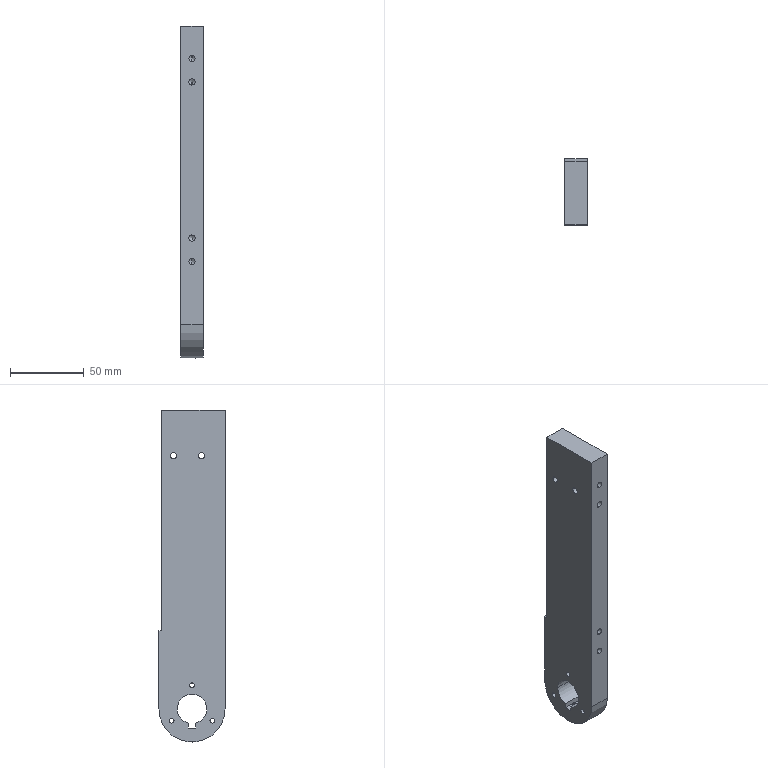Component | SolidWorks | 04-1 | 1 solid | 54 faces | box 15 x 45 x 225.5 mm | volume 137244 mm3 | cylinder 30 | cone 14 | plane 10 | commonest cylinder face diameters 4.2 x20 3.3 x6 20 x3 45 x1
build123d program:
from build123d import *

# Parameters (mm, degrees)
SKETCH1_W             = 203
SKETCH1_H             = 45
EXTRUDE1_DEPTH        = 7.5
SKETCH2_R             = 22.5
EXTRUDE2_DEPTH        = 15
SKETCH4_R             = 10
EXTRUDE3_DEPTH        = 127.914
SKETCH5_W             = 150
SKETCH5_H             = 15
CUT_EXTRUDE1_DEPTH    = 2
SKETCH6_W             = 7
SKETCH6_H             = 5
EXTRUDE4_DEPTH        = 127.914
M5_TAPPED_HOLE1_D     = 4.2
M5_TAPPED_HOLE1_DEPTH = 14
M5_TAPPED_HOLE1_TIP   = 1.262
M5_TAPPED_HOLE2_D     = 4.2
M5_TAPPED_HOLE2_DEPTH = 14
M5_TAPPED_HOLE2_TIP   = 1.262
M4_TAPPED_HOLE1_D     = 3.3
M5_TAPPED_HOLE3_D     = 4.2
M5_TAPPED_HOLE4_D     = 4.2
M5_TAPPED_HOLE4_DEPTH = 12.4
M5_TAPPED_HOLE4_TIP   = 1.262


with BuildPart() as part:
    # Sketch1 → Extrude1 (new, symmetric)
    with BuildSketch(Plane(origin=(0, 0, 0), x_dir=(1, 0, 0), z_dir=(0, 1, 0))):
        Rectangle(SKETCH1_W, SKETCH1_H)
    extrude(amount=EXTRUDE1_DEPTH, both=True)

    # Sketch2 → Extrude2 (add)
    with BuildSketch(Plane(origin=(0, 7.5, 0), x_dir=(1, 0, 0), z_dir=(0, 1, 0))):
        with Locations((101.5, 0)):
            Circle(SKETCH2_R)
    extrude(amount=-EXTRUDE2_DEPTH)

    # Sketch4 → Extrude3 (cut, through all)
    with BuildSketch(Plane(origin=(0, 7.5, 0), x_dir=(1, 0, 0), z_dir=(0, 1, 0))):
        with Locations(Location((101.5, 0, 0), (0, 0, 270))):
            Circle(SKETCH4_R)
    extrude(amount=-EXTRUDE3_DEPTH, mode=Mode.SUBTRACT)

    # Sketch5 → Cut-Extrude1 (cut)
    with BuildSketch(Plane(origin=(0, 0, -22.5), x_dir=(-1, 0, 0), z_dir=(0, 0, -1))):
        with Locations((26.5, 0)):
            Rectangle(SKETCH5_W, SKETCH5_H)
    extrude(amount=-CUT_EXTRUDE1_DEPTH, mode=Mode.SUBTRACT)

    # Sketch6 → Extrude4 (cut, through all)
    with BuildSketch(Plane(origin=(0, 7.5, 0), x_dir=(1, 0, 0), z_dir=(0, 1, 0))):
        with Locations((111, 0)):
            Rectangle(SKETCH6_W, SKETCH6_H)
    extrude(amount=-EXTRUDE4_DEPTH, mode=Mode.SUBTRACT)

    # M5 Tapped Hole1
    with Locations(Plane.XY.offset(22.5)):
        with Locations((-79.5, 0), (-63.5, 0), (42.5, 0), (58.5, 0)):
            Hole(M5_TAPPED_HOLE1_D / 2, depth=M5_TAPPED_HOLE1_DEPTH)
            with Locations((0, 0, -(M5_TAPPED_HOLE1_DEPTH + M5_TAPPED_HOLE1_TIP / 2))):  # 118° drill point
                Cone(0, M5_TAPPED_HOLE1_D / 2, M5_TAPPED_HOLE1_TIP, mode=Mode.SUBTRACT)

    # M5 Tapped Hole2
    with Locations(Plane.ZY.offset(-114.5)):
        with Locations((0, 0)):
            Hole(M5_TAPPED_HOLE2_D / 2, depth=M5_TAPPED_HOLE2_DEPTH)
            with Locations((0, 0, -(M5_TAPPED_HOLE2_DEPTH + M5_TAPPED_HOLE2_TIP / 2))):  # 118° drill point
                Cone(0, M5_TAPPED_HOLE2_D / 2, M5_TAPPED_HOLE2_TIP, mode=Mode.SUBTRACT)

    # M4 Tapped Hole1 (through all)
    with Locations(Plane(origin=(0, 7.5, 0), x_dir=(1, 0, 0), z_dir=(0, 1, 0))):
        with Locations((85.5, 0), (109.5, 13.856), (109.5, -13.856)):
            Hole(M4_TAPPED_HOLE1_D / 2)

    # M5 Tapped Hole3 (through all)
    with Locations(Plane(origin=(0, -7.5, 0), x_dir=(-1, 0, 0), z_dir=(0, -1, 0))):
        with Locations((70.5, 12.5), (70.5, -6.5)):
            Hole(M5_TAPPED_HOLE3_D / 2)

    # M5 Tapped Hole4
    with Locations(Plane(origin=(0, 0, -20.5), x_dir=(-1, 0, 0), z_dir=(0, 0, -1))):
        with Locations((86.5, 0), (26.5, 0), (-33.5, 0), (86.5, -156), (26.5, -156), (-33.5, -156)):
            Hole(M5_TAPPED_HOLE4_D / 2, depth=M5_TAPPED_HOLE4_DEPTH)
            with Locations((0, 0, -(M5_TAPPED_HOLE4_DEPTH + M5_TAPPED_HOLE4_TIP / 2))):  # 118° drill point
                Cone(0, M5_TAPPED_HOLE4_D / 2, M5_TAPPED_HOLE4_TIP, mode=Mode.SUBTRACT)


solid = part.part

# Placed as in the assembly
solid = solid.moved(Location((-70, -32.5, 131.5), (90, 0, -90)))